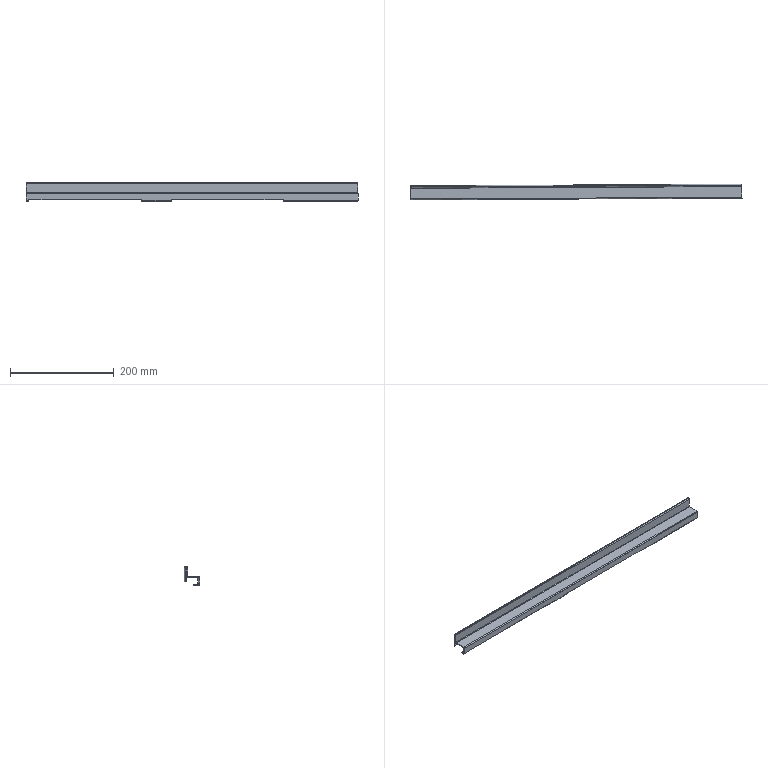Component | SolidWorks | RAY MONTAJ-1_RAY SA-2 | 1 solid | 63 faces | volume 55612 mm3 | plane 49 | cylinder 14 | commonest cylinder face diameters 1.473 x7 3.473 x7